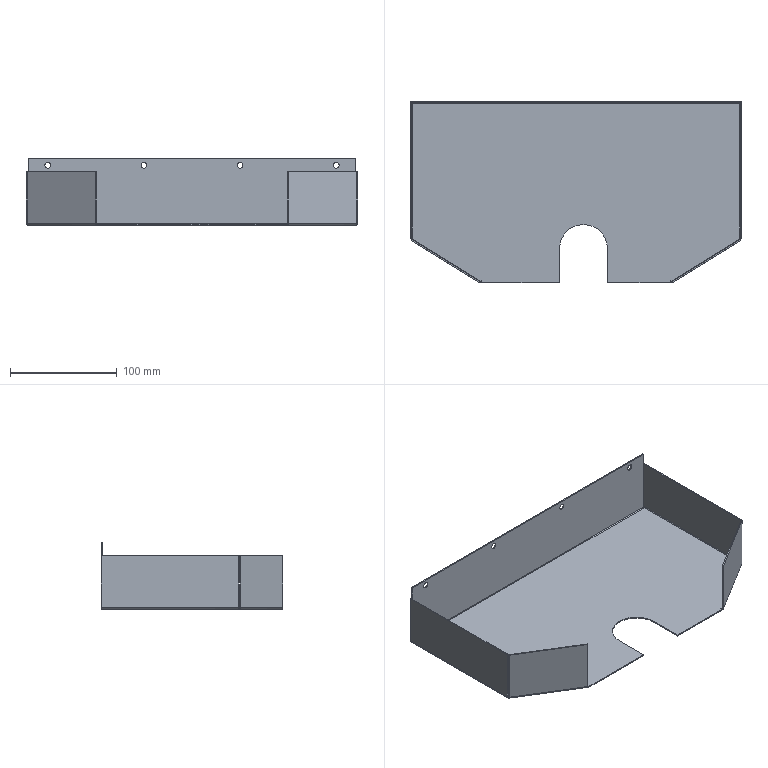Component | SolidWorks | LD101-02--Q1072-Q1-2-1 | 1 solid | 68 faces | volume 86080 mm3 | plane 45 | cylinder 19 | spline 4 | commonest cylinder face diameters 5.5 x8 3.473 x5 1.473 x5 45 x1 | material SUS304